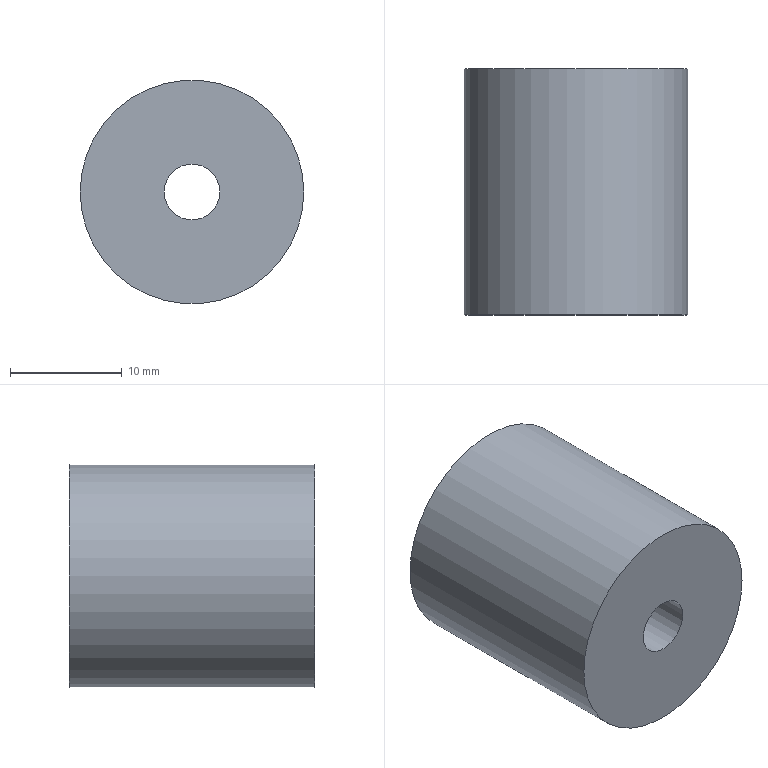Component | NX | BUSHING_6 | 1 solid | 4 faces | box 20 x 22 x 20 mm | volume 6480 mm3 | cylinder 2 | plane 2 | commonest cylinder face diameters 20 x1 5 x1
STEP:
#1=CARTESIAN_POINT('',(0.,0.,0.));
#2=DIRECTION('',(0.,0.,1.));
#3=DIRECTION('',(1.,0.,0.));
#4=AXIS2_PLACEMENT_3D('',#1,#2,#3);
#5=CARTESIAN_POINT('',(1444.254,1145.,813.574));
#6=VERTEX_POINT('',#5);
#7=CARTESIAN_POINT('',(1434.254,1145.,813.574));
#8=DIRECTION('',(0.,1.,0.));
#9=DIRECTION('',(1.,0.,0.));
#10=AXIS2_PLACEMENT_3D('',#7,#8,#9);
#11=CIRCLE('',#10,10.);
#12=CARTESIAN_POINT('',(1434.254,1145.,813.574));
#13=DIRECTION('',(0.,-1.,0.));
#14=DIRECTION('',(0.,0.,-1.));
#15=AXIS2_PLACEMENT_3D('',#12,#13,#14);
#16=CYLINDRICAL_SURFACE('',#15,10.);
#17=CARTESIAN_POINT('',(7.854,0.));
#18=DIRECTION('',(-1.,0.));
#19=VECTOR('',#18,1.);
#20=LINE('',#17,#19);
#21=(GEOMETRIC_REPRESENTATION_CONTEXT(2)PARAMETRIC_REPRESENTATION_CONTEXT()REPRESENTATION_CONTEXT('',''));
#22=DEFINITIONAL_REPRESENTATION('',(#20),#21);
#23=PCURVE('',#16,#22);
#24=CARTESIAN_POINT('',(1434.254,1145.,813.574));
#25=DIRECTION('',(0.,1.,0.));
#26=DIRECTION('',(0.,0.,1.));
#27=AXIS2_PLACEMENT_3D('',#24,#25,#26);
#28=PLANE('',#27);
#29=CARTESIAN_POINT('',(0.,0.));
#30=DIRECTION('',(0.,1.));
#31=AXIS2_PLACEMENT_2D('',#29,#30);
#32=CIRCLE('',#31,10.);
#33=(GEOMETRIC_REPRESENTATION_CONTEXT(2)PARAMETRIC_REPRESENTATION_CONTEXT()REPRESENTATION_CONTEXT('',''));
#34=DEFINITIONAL_REPRESENTATION('',(#32),#33);
#35=PCURVE('',#28,#34);
#36=SURFACE_CURVE('',#11,(#23,#35),.PCURVE_S1.);
#37=EDGE_CURVE('',#6,#6,#36,.T.);
#38=ORIENTED_EDGE('',*,*,#37,.F.);
#39=CARTESIAN_POINT('',(1444.254,1123.,813.574));
#40=VERTEX_POINT('',#39);
#41=CARTESIAN_POINT('',(1444.254,1145.,813.574));
#42=CARTESIAN_POINT('',(1444.254,1123.,813.574));
#43=B_SPLINE_CURVE_WITH_KNOTS('',1,(#41,#42),.UNSPECIFIED.,.F.,.F.,(2,2),(0.,22.),.PIECEWISE_BEZIER_KNOTS.);
#44=CARTESIAN_POINT('',(7.854,0.));
#45=DIRECTION('',(0.,1.));
#46=VECTOR('',#45,1.);
#47=LINE('',#44,#46);
#48=(GEOMETRIC_REPRESENTATION_CONTEXT(2)PARAMETRIC_REPRESENTATION_CONTEXT()REPRESENTATION_CONTEXT('',''));
#49=DEFINITIONAL_REPRESENTATION('',(#47),#48);
#50=PCURVE('',#16,#49);
#51=CARTESIAN_POINT('',(1.571,0.));
#52=DIRECTION('',(0.,1.));
#53=VECTOR('',#52,1.);
#54=LINE('',#51,#53);
#55=(GEOMETRIC_REPRESENTATION_CONTEXT(2)PARAMETRIC_REPRESENTATION_CONTEXT()REPRESENTATION_CONTEXT('',''));
#56=DEFINITIONAL_REPRESENTATION('',(#54),#55);
#57=PCURVE('',#16,#56);
#58=SEAM_CURVE('',#43,(#50,#57),.PCURVE_S1.);
#59=EDGE_CURVE('',#6,#40,#58,.T.);
#60=ORIENTED_EDGE('',*,*,#59,.T.);
#61=CARTESIAN_POINT('',(1434.254,1123.,813.574));
#62=DIRECTION('',(0.,1.,0.));
#63=DIRECTION('',(1.,0.,0.));
#64=AXIS2_PLACEMENT_3D('',#61,#62,#63);
#65=CIRCLE('',#64,10.);
#66=CARTESIAN_POINT('',(7.854,22.));
#67=DIRECTION('',(-1.,0.));
#68=VECTOR('',#67,1.);
#69=LINE('',#66,#68);
#70=(GEOMETRIC_REPRESENTATION_CONTEXT(2)PARAMETRIC_REPRESENTATION_CONTEXT()REPRESENTATION_CONTEXT('',''));
#71=DEFINITIONAL_REPRESENTATION('',(#69),#70);
#72=PCURVE('',#16,#71);
#73=CARTESIAN_POINT('',(1434.254,1123.,813.574));
#74=DIRECTION('',(0.,1.,0.));
#75=DIRECTION('',(0.,0.,1.));
#76=AXIS2_PLACEMENT_3D('',#73,#74,#75);
#77=PLANE('',#76);
#78=CARTESIAN_POINT('',(0.,0.));
#79=DIRECTION('',(0.,1.));
#80=AXIS2_PLACEMENT_2D('',#78,#79);
#81=CIRCLE('',#80,10.);
#82=(GEOMETRIC_REPRESENTATION_CONTEXT(2)PARAMETRIC_REPRESENTATION_CONTEXT()REPRESENTATION_CONTEXT('',''));
#83=DEFINITIONAL_REPRESENTATION('',(#81),#82);
#84=PCURVE('',#77,#83);
#85=SURFACE_CURVE('',#65,(#72,#84),.PCURVE_S1.);
#86=EDGE_CURVE('',#40,#40,#85,.T.);
#87=ORIENTED_EDGE('',*,*,#86,.T.);
#88=ORIENTED_EDGE('',*,*,#59,.F.);
#89=EDGE_LOOP('',(#38,#60,#87,#88));
#90=FACE_BOUND('',#89,.T.);
#91=ADVANCED_FACE('',(#90),#16,.T.);
#92=CARTESIAN_POINT('',(1436.754,1145.,813.574));
#93=VERTEX_POINT('',#92);
#94=CARTESIAN_POINT('',(1434.254,1145.,813.574));
#95=DIRECTION('',(0.,1.,0.));
#96=DIRECTION('',(1.,0.,0.));
#97=AXIS2_PLACEMENT_3D('',#94,#95,#96);
#98=CIRCLE('',#97,2.5);
#99=CARTESIAN_POINT('',(1434.254,1145.,813.574));
#100=DIRECTION('',(0.,-1.,0.));
#101=DIRECTION('',(0.,0.,-1.));
#102=AXIS2_PLACEMENT_3D('',#99,#100,#101);
#103=CYLINDRICAL_SURFACE('',#102,2.5);
#104=CARTESIAN_POINT('',(7.854,0.));
#105=DIRECTION('',(-1.,0.));
#106=VECTOR('',#105,1.);
#107=LINE('',#104,#106);
#108=(GEOMETRIC_REPRESENTATION_CONTEXT(2)PARAMETRIC_REPRESENTATION_CONTEXT()REPRESENTATION_CONTEXT('',''));
#109=DEFINITIONAL_REPRESENTATION('',(#107),#108);
#110=PCURVE('',#103,#109);
#111=CARTESIAN_POINT('',(0.,0.));
#112=DIRECTION('',(0.,1.));
#113=AXIS2_PLACEMENT_2D('',#111,#112);
#114=CIRCLE('',#113,2.5);
#115=(GEOMETRIC_REPRESENTATION_CONTEXT(2)PARAMETRIC_REPRESENTATION_CONTEXT()REPRESENTATION_CONTEXT('',''));
#116=DEFINITIONAL_REPRESENTATION('',(#114),#115);
#117=PCURVE('',#28,#116);
#118=SURFACE_CURVE('',#98,(#110,#117),.PCURVE_S1.);
#119=EDGE_CURVE('',#93,#93,#118,.T.);
#120=ORIENTED_EDGE('',*,*,#119,.F.);
#121=CARTESIAN_POINT('',(1436.754,1123.,813.574));
#122=VERTEX_POINT('',#121);
#123=CARTESIAN_POINT('',(1436.754,1145.,813.574));
#124=CARTESIAN_POINT('',(1436.754,1123.,813.574));
#125=B_SPLINE_CURVE_WITH_KNOTS('',1,(#123,#124),.UNSPECIFIED.,.F.,.F.,(2,2),(0.,22.),.PIECEWISE_BEZIER_KNOTS.);
#126=CARTESIAN_POINT('',(7.854,0.));
#127=DIRECTION('',(0.,1.));
#128=VECTOR('',#127,1.);
#129=LINE('',#126,#128);
#130=(GEOMETRIC_REPRESENTATION_CONTEXT(2)PARAMETRIC_REPRESENTATION_CONTEXT()REPRESENTATION_CONTEXT('',''));
#131=DEFINITIONAL_REPRESENTATION('',(#129),#130);
#132=PCURVE('',#103,#131);
#133=CARTESIAN_POINT('',(1.571,0.));
#134=DIRECTION('',(0.,1.));
#135=VECTOR('',#134,1.);
#136=LINE('',#133,#135);
#137=(GEOMETRIC_REPRESENTATION_CONTEXT(2)PARAMETRIC_REPRESENTATION_CONTEXT()REPRESENTATION_CONTEXT('',''));
#138=DEFINITIONAL_REPRESENTATION('',(#136),#137);
#139=PCURVE('',#103,#138);
#140=SEAM_CURVE('',#125,(#132,#139),.PCURVE_S1.);
#141=EDGE_CURVE('',#93,#122,#140,.T.);
#142=ORIENTED_EDGE('',*,*,#141,.T.);
#143=CARTESIAN_POINT('',(1434.254,1123.,813.574));
#144=DIRECTION('',(0.,1.,0.));
#145=DIRECTION('',(1.,0.,0.));
#146=AXIS2_PLACEMENT_3D('',#143,#144,#145);
#147=CIRCLE('',#146,2.5);
#148=CARTESIAN_POINT('',(7.854,22.));
#149=DIRECTION('',(-1.,0.));
#150=VECTOR('',#149,1.);
#151=LINE('',#148,#150);
#152=(GEOMETRIC_REPRESENTATION_CONTEXT(2)PARAMETRIC_REPRESENTATION_CONTEXT()REPRESENTATION_CONTEXT('',''));
#153=DEFINITIONAL_REPRESENTATION('',(#151),#152);
#154=PCURVE('',#103,#153);
#155=CARTESIAN_POINT('',(0.,0.));
#156=DIRECTION('',(0.,1.));
#157=AXIS2_PLACEMENT_2D('',#155,#156);
#158=CIRCLE('',#157,2.5);
#159=(GEOMETRIC_REPRESENTATION_CONTEXT(2)PARAMETRIC_REPRESENTATION_CONTEXT()REPRESENTATION_CONTEXT('',''));
#160=DEFINITIONAL_REPRESENTATION('',(#158),#159);
#161=PCURVE('',#77,#160);
#162=SURFACE_CURVE('',#147,(#154,#161),.PCURVE_S1.);
#163=EDGE_CURVE('',#122,#122,#162,.T.);
#164=ORIENTED_EDGE('',*,*,#163,.T.);
#165=ORIENTED_EDGE('',*,*,#141,.F.);
#166=EDGE_LOOP('',(#120,#142,#164,#165));
#167=FACE_BOUND('',#166,.F.);
#168=ADVANCED_FACE('',(#167),#103,.F.);
#169=ORIENTED_EDGE('',*,*,#37,.T.);
#170=EDGE_LOOP('',(#169));
#171=FACE_BOUND('',#170,.T.);
#172=ORIENTED_EDGE('',*,*,#119,.F.);
#173=EDGE_LOOP('',(#172));
#174=FACE_BOUND('',#173,.T.);
#175=ADVANCED_FACE('',(#171,#174),#28,.T.);
#176=ORIENTED_EDGE('',*,*,#86,.F.);
#177=EDGE_LOOP('',(#176));
#178=FACE_BOUND('',#177,.T.);
#179=ORIENTED_EDGE('',*,*,#163,.T.);
#180=EDGE_LOOP('',(#179));
#181=FACE_BOUND('',#180,.T.);
#182=ADVANCED_FACE('',(#178,#181),#77,.F.);
#183=CLOSED_SHELL('',(#91,#168,#175,#182));
#184=MANIFOLD_SOLID_BREP('',#183);
#185=(LENGTH_UNIT()NAMED_UNIT(*)SI_UNIT(.MILLI.,.METRE.));
#186=UNCERTAINTY_MEASURE_WITH_UNIT(LENGTH_MEASURE(0.00001),#185,'','');
#187=(NAMED_UNIT(*)PLANE_ANGLE_UNIT()SI_UNIT($,.RADIAN.));
#188=(NAMED_UNIT(*)SI_UNIT($,.STERADIAN.)SOLID_ANGLE_UNIT());
#189=(GEOMETRIC_REPRESENTATION_CONTEXT(3)GLOBAL_UNCERTAINTY_ASSIGNED_CONTEXT((#186))GLOBAL_UNIT_ASSIGNED_CONTEXT((#185,#187,#188))REPRESENTATION_CONTEXT('',''));
#190=ADVANCED_BREP_SHAPE_REPRESENTATION('',(#4,#184),#189);